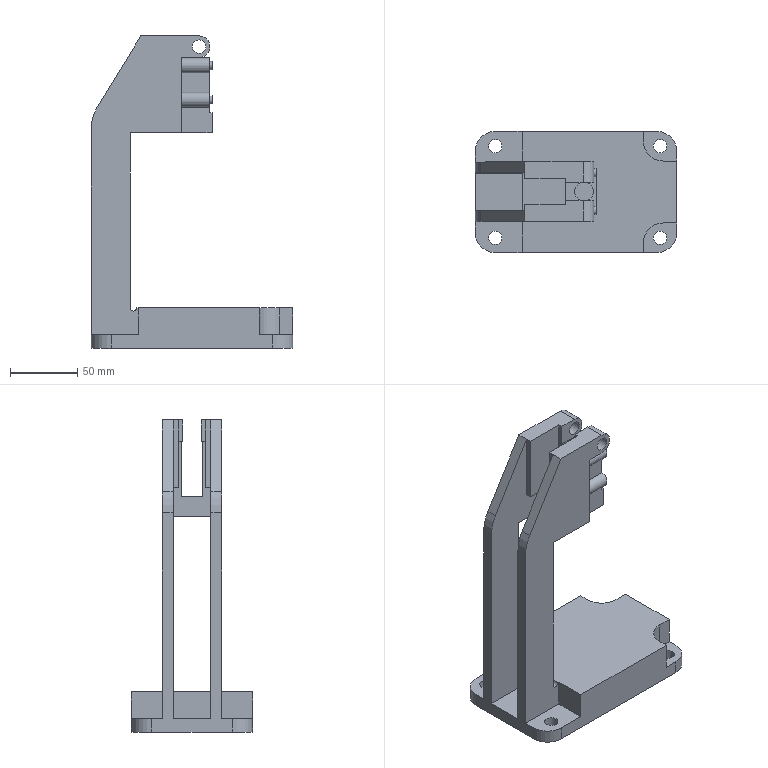Component | NX | MACHINE_BASE | 2 solids | 91 faces | volume 489286 mm3 | plane 64 | cylinder 27 | commonest cylinder face diameters 30 x6 10 x6 11 x4 6 x4 16 x2 60 x2 5 x2 14 x1